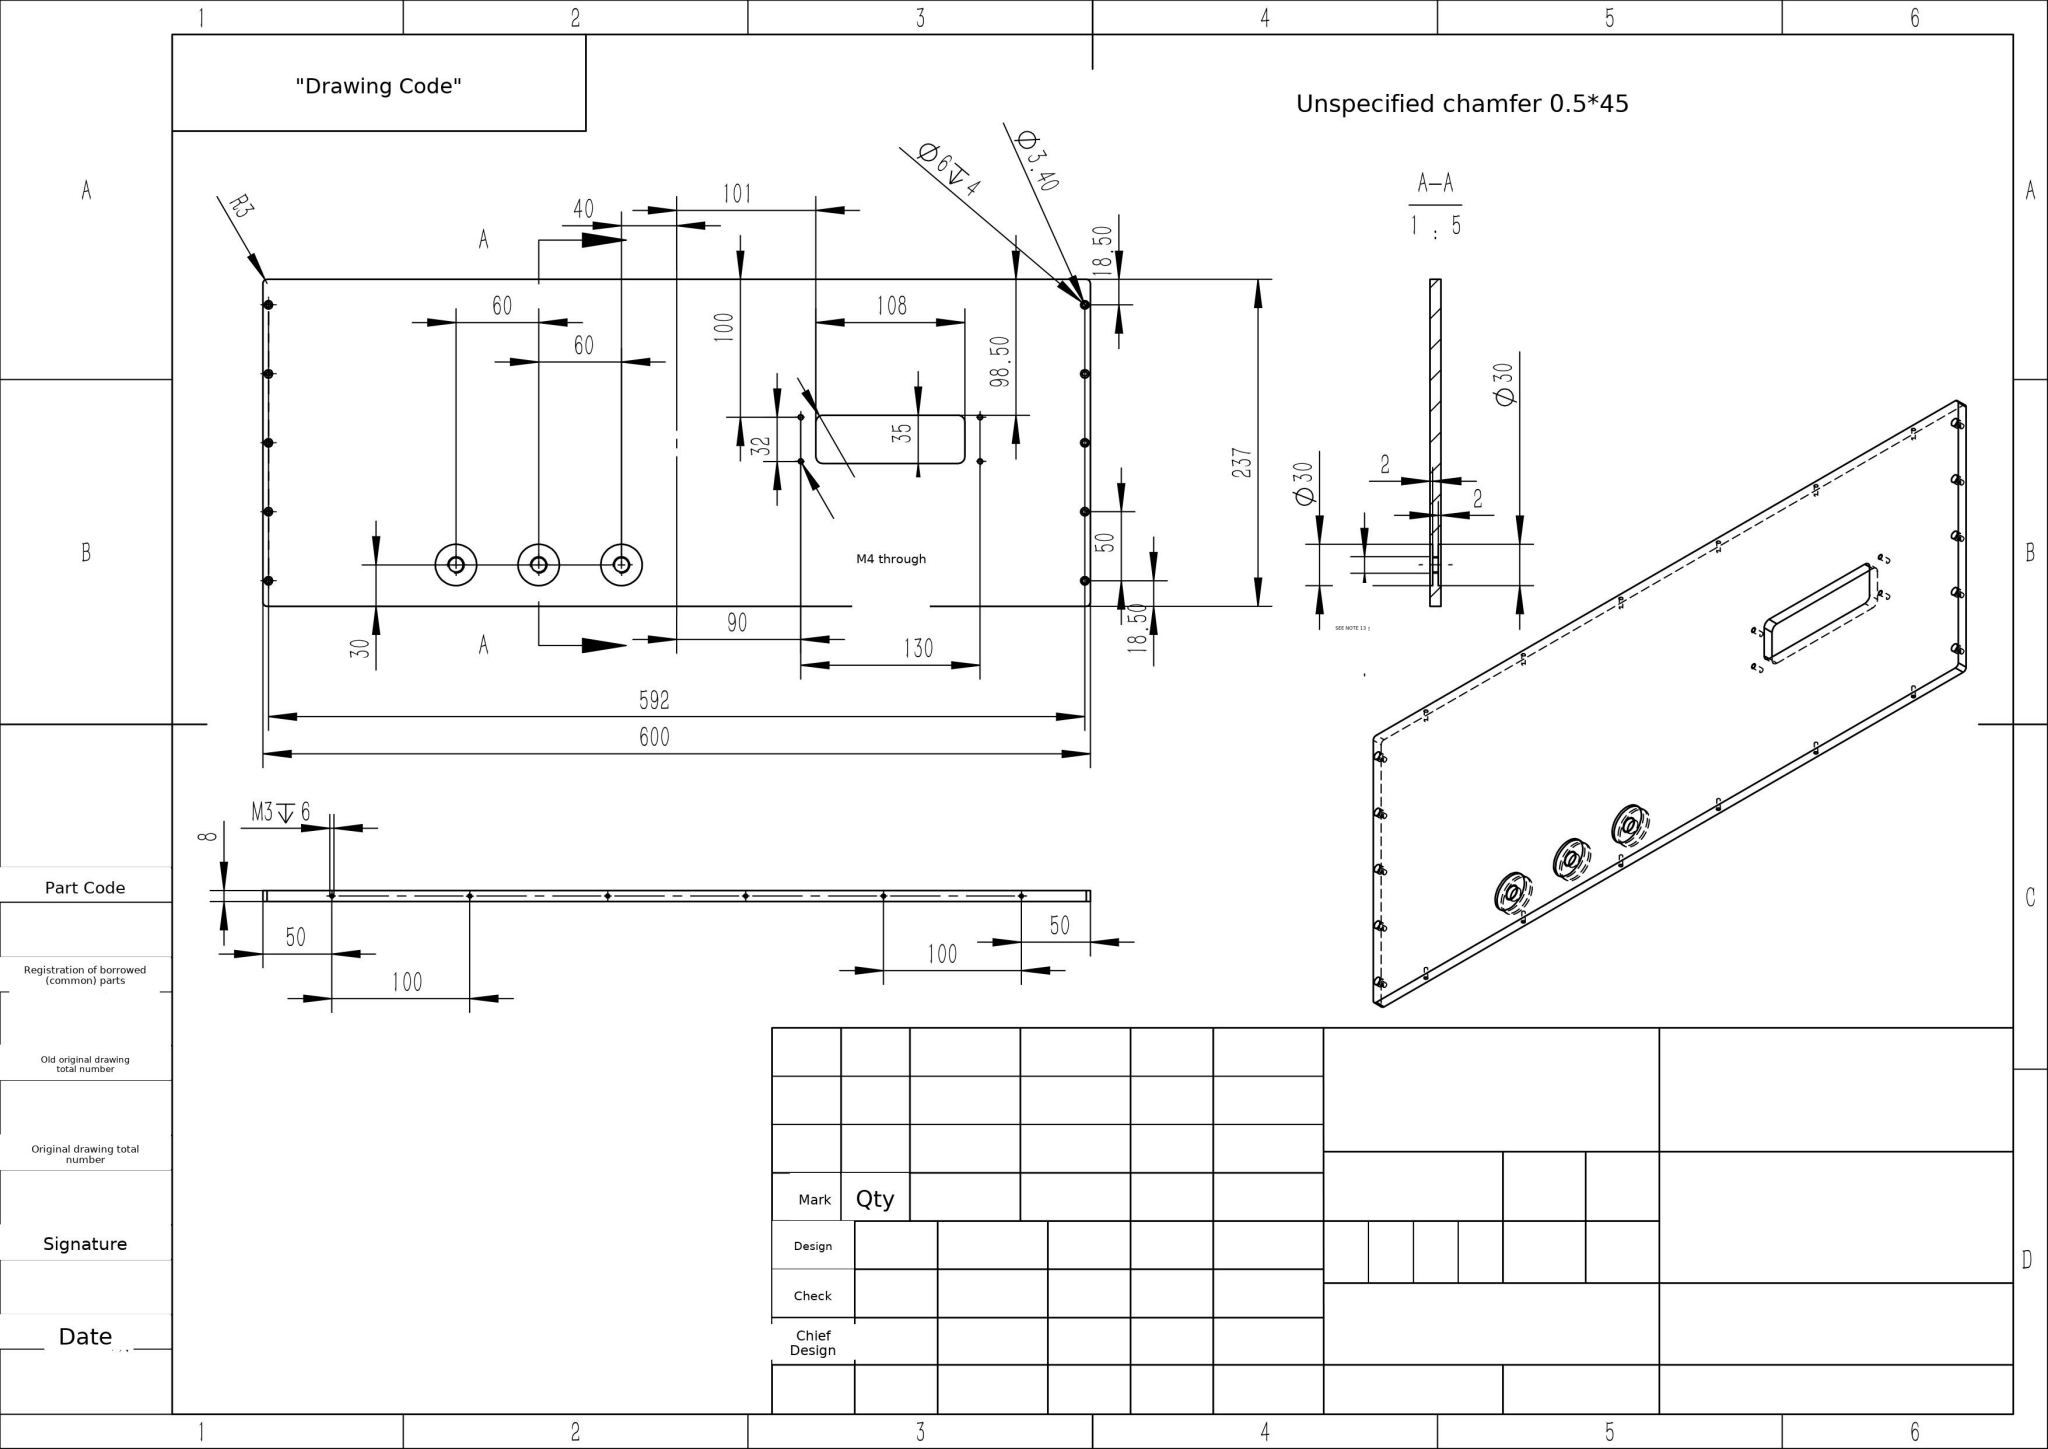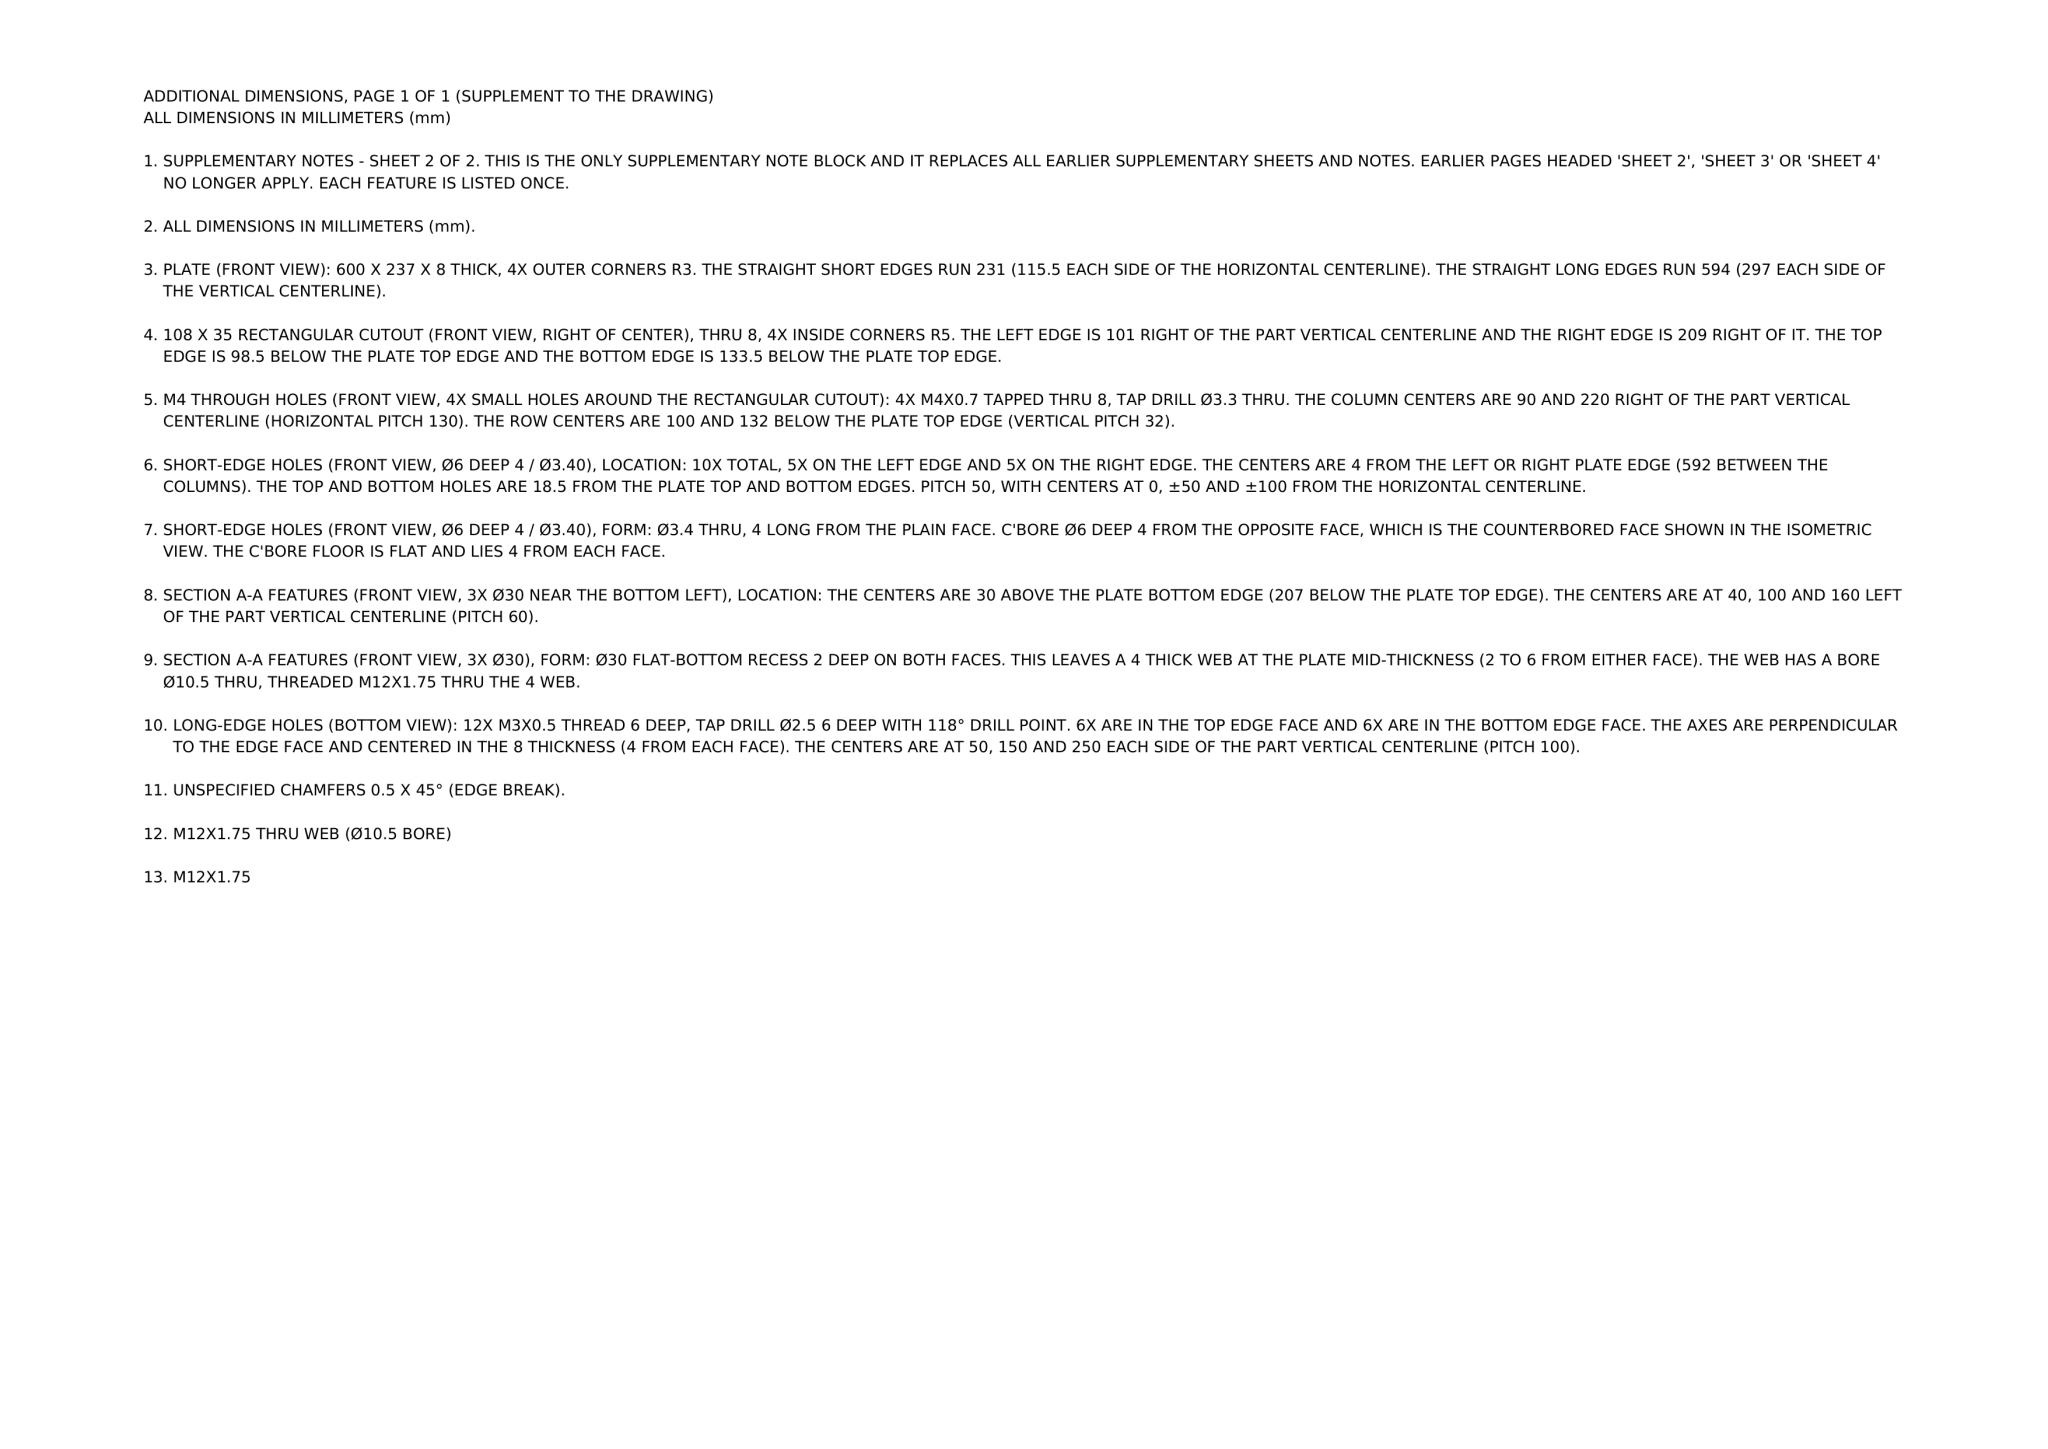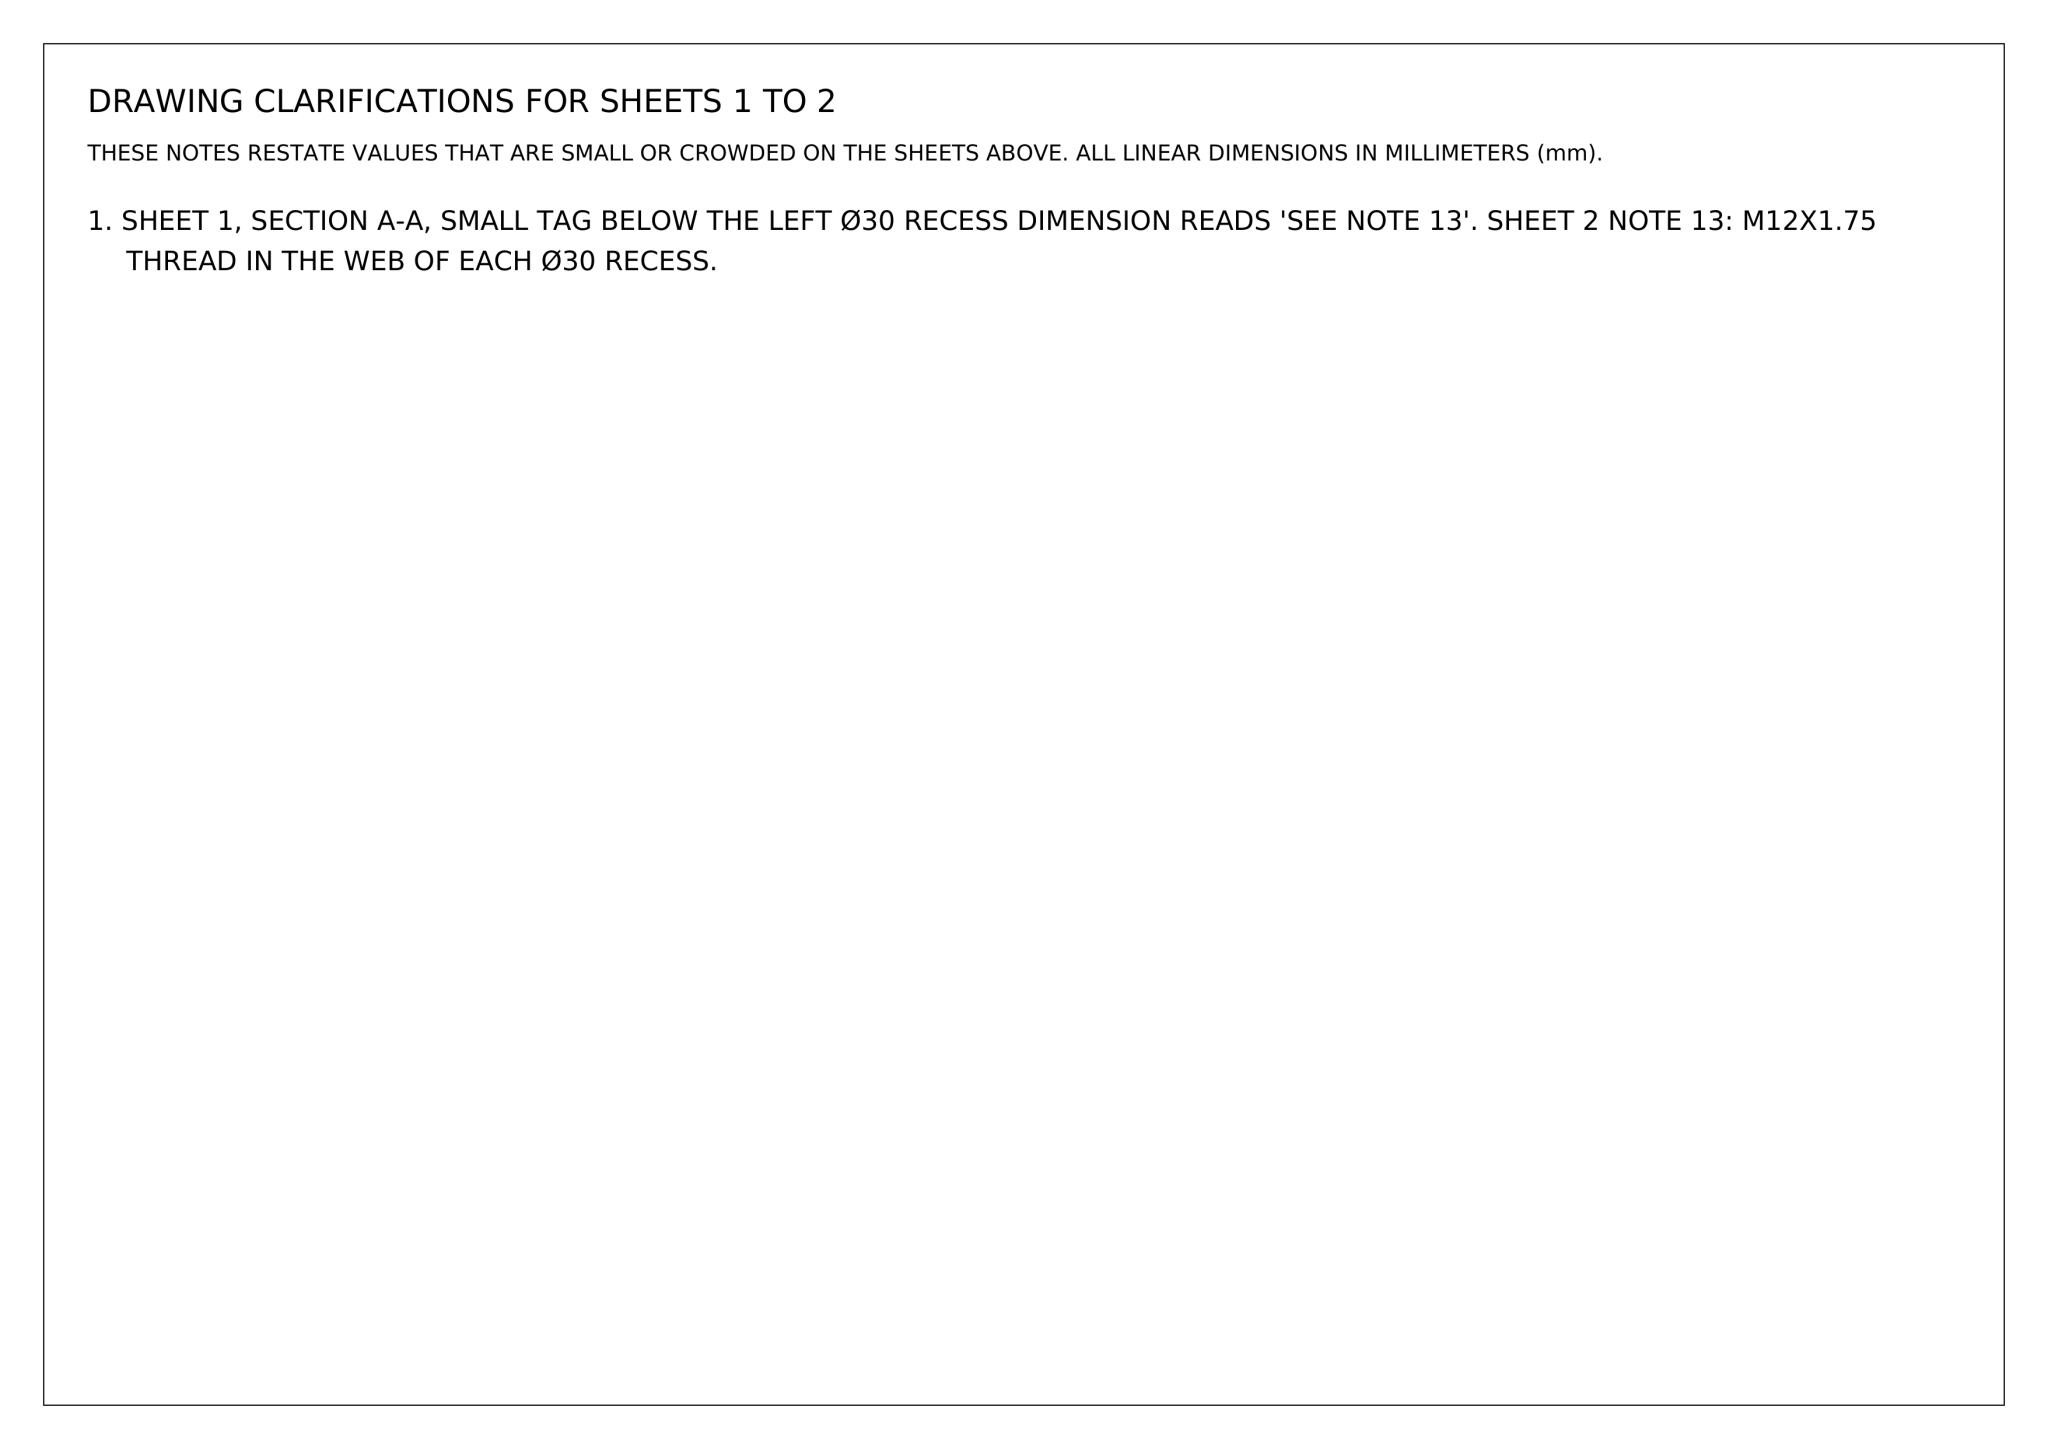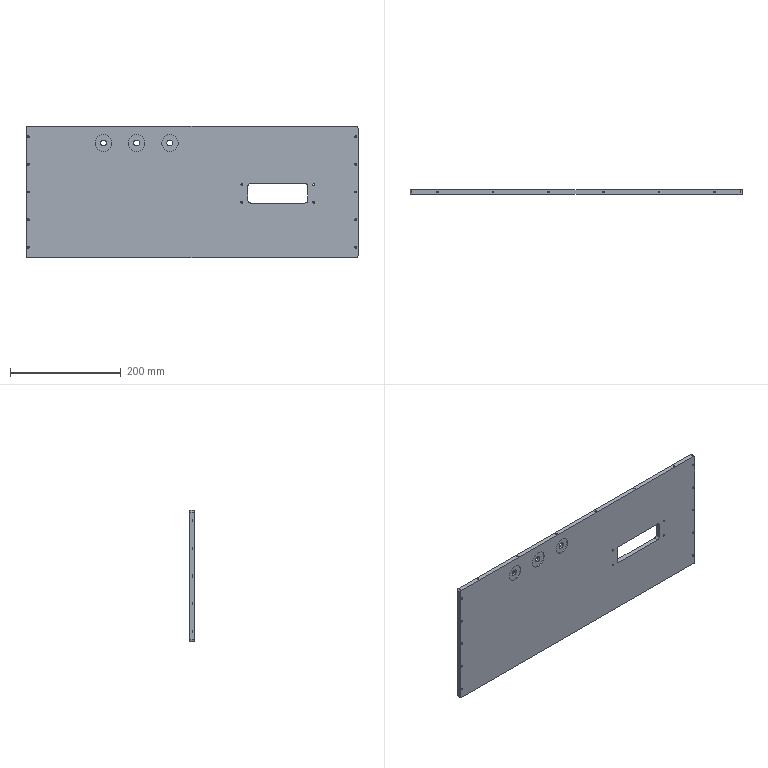Part | NX | mm | 1 solid | 148 faces | box 600 x 8 x 237 mm | volume 1095665 mm3 | cylinder 98 | plane 26 | cone 24 | commonest cylinder face diameters 2.5 x24 6 x24 3.4 x20 30 x12 3.3 x8 10.5 x6 10 x4